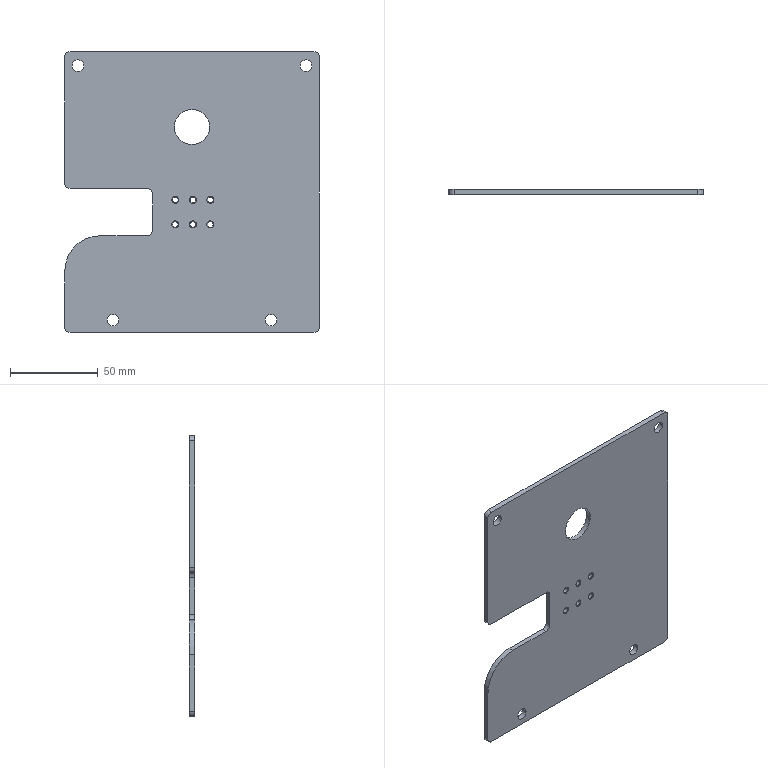Component | SolidWorks | QX1-23-BJCoverPlate-1 | 1 solid | 52 faces | volume 63763 mm3 | cylinder 30 | cone 12 | plane 10 | commonest cylinder face diameters 3.3 x12 6.6 x8 6 x7 20 x2 40 x1 | material Q235